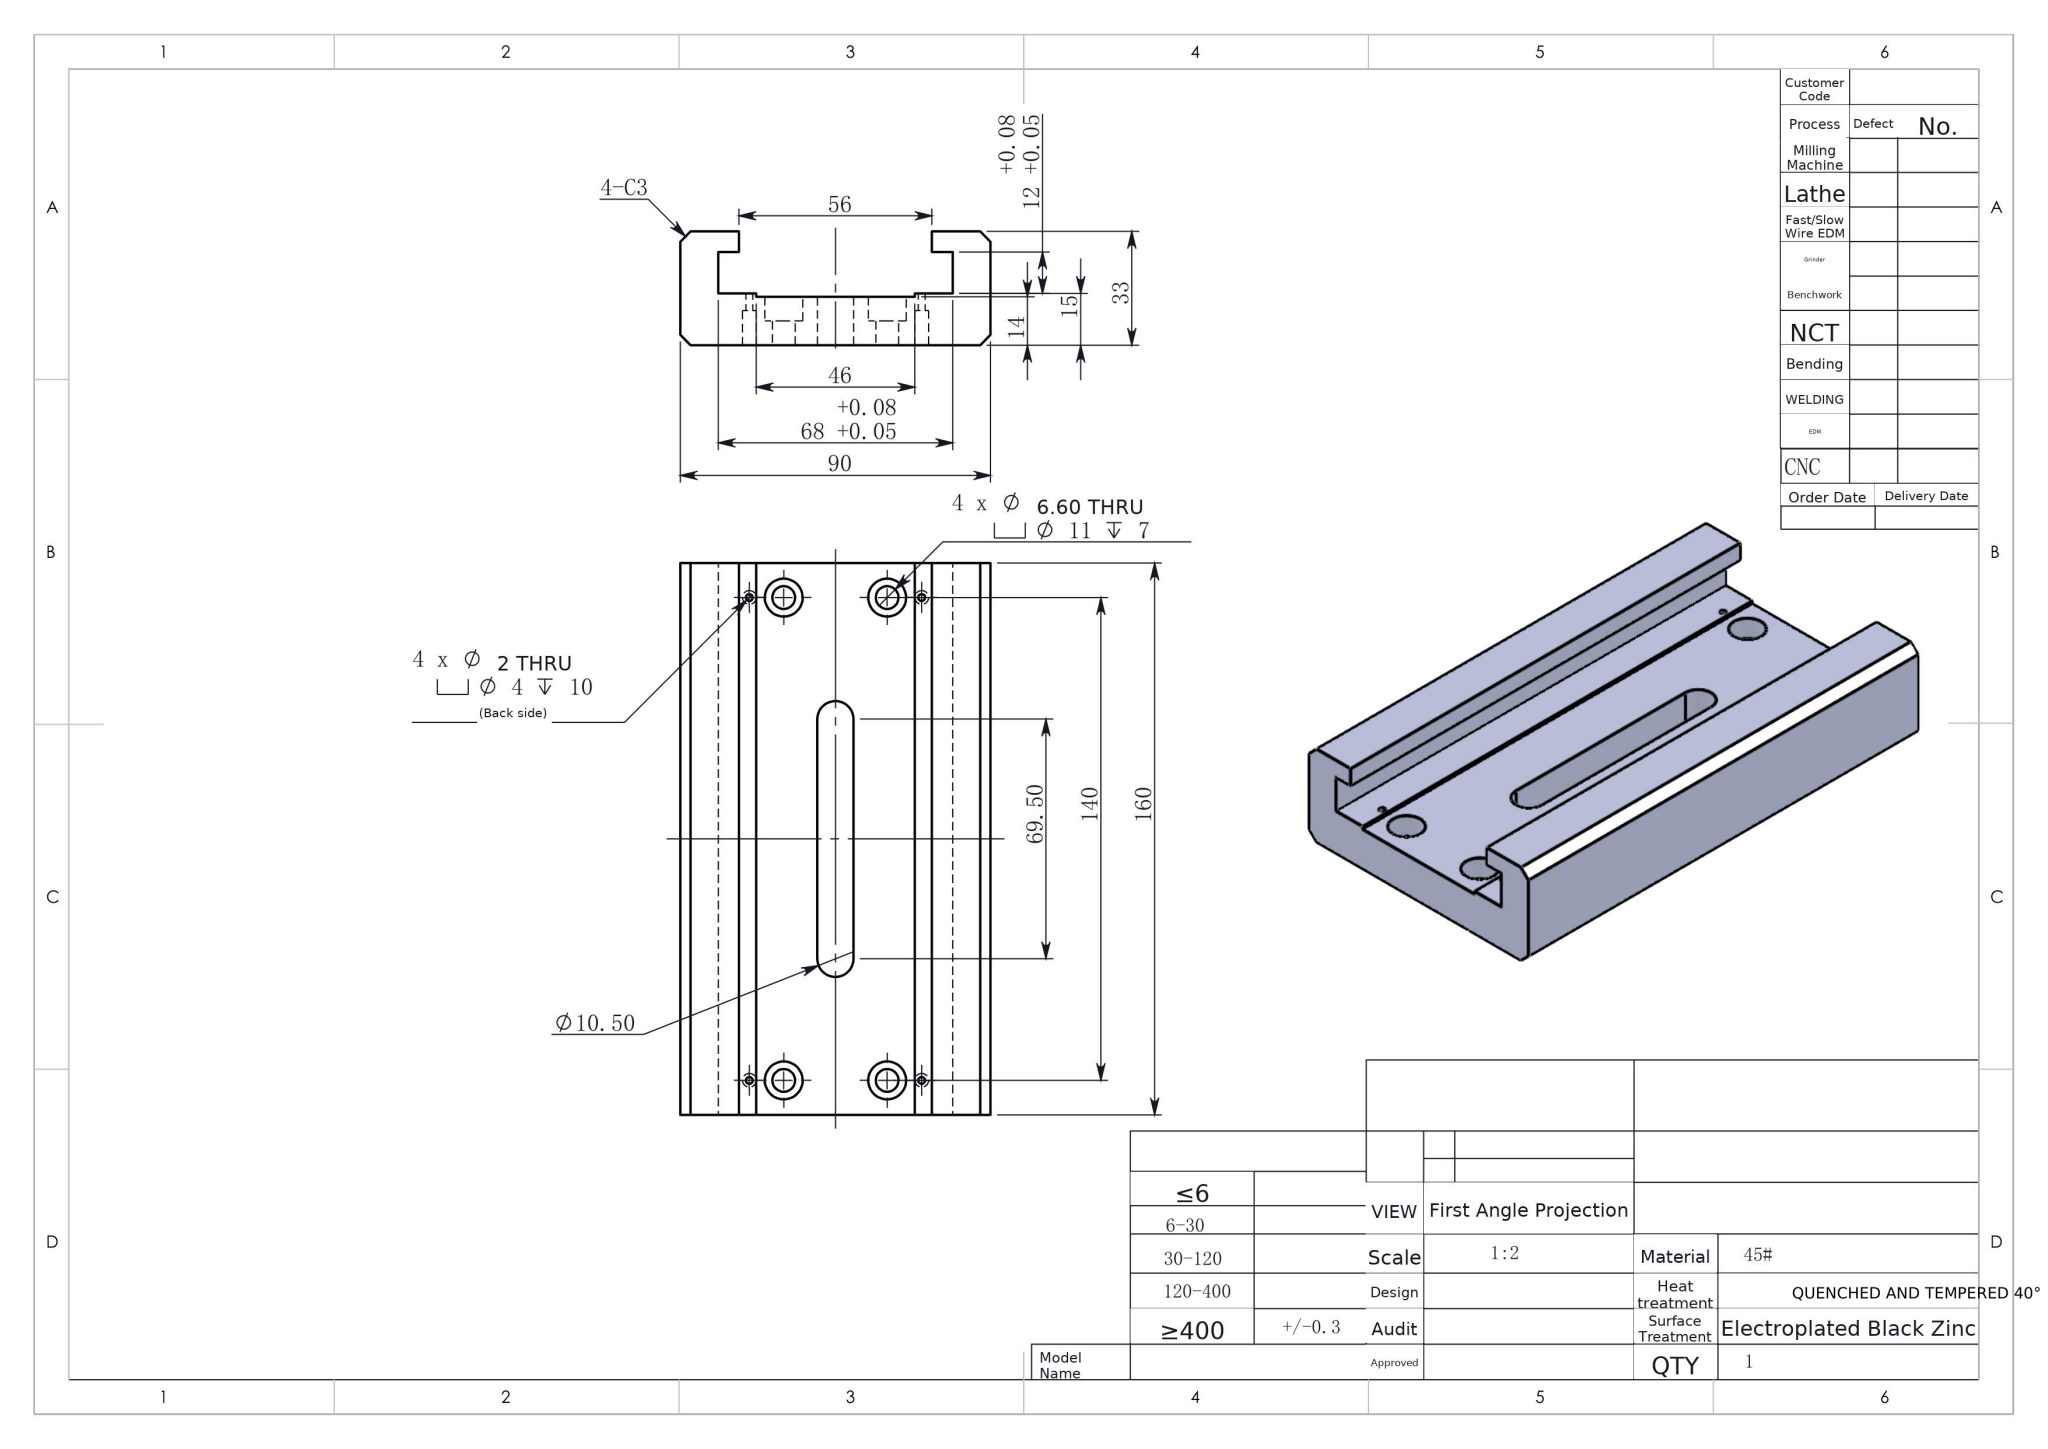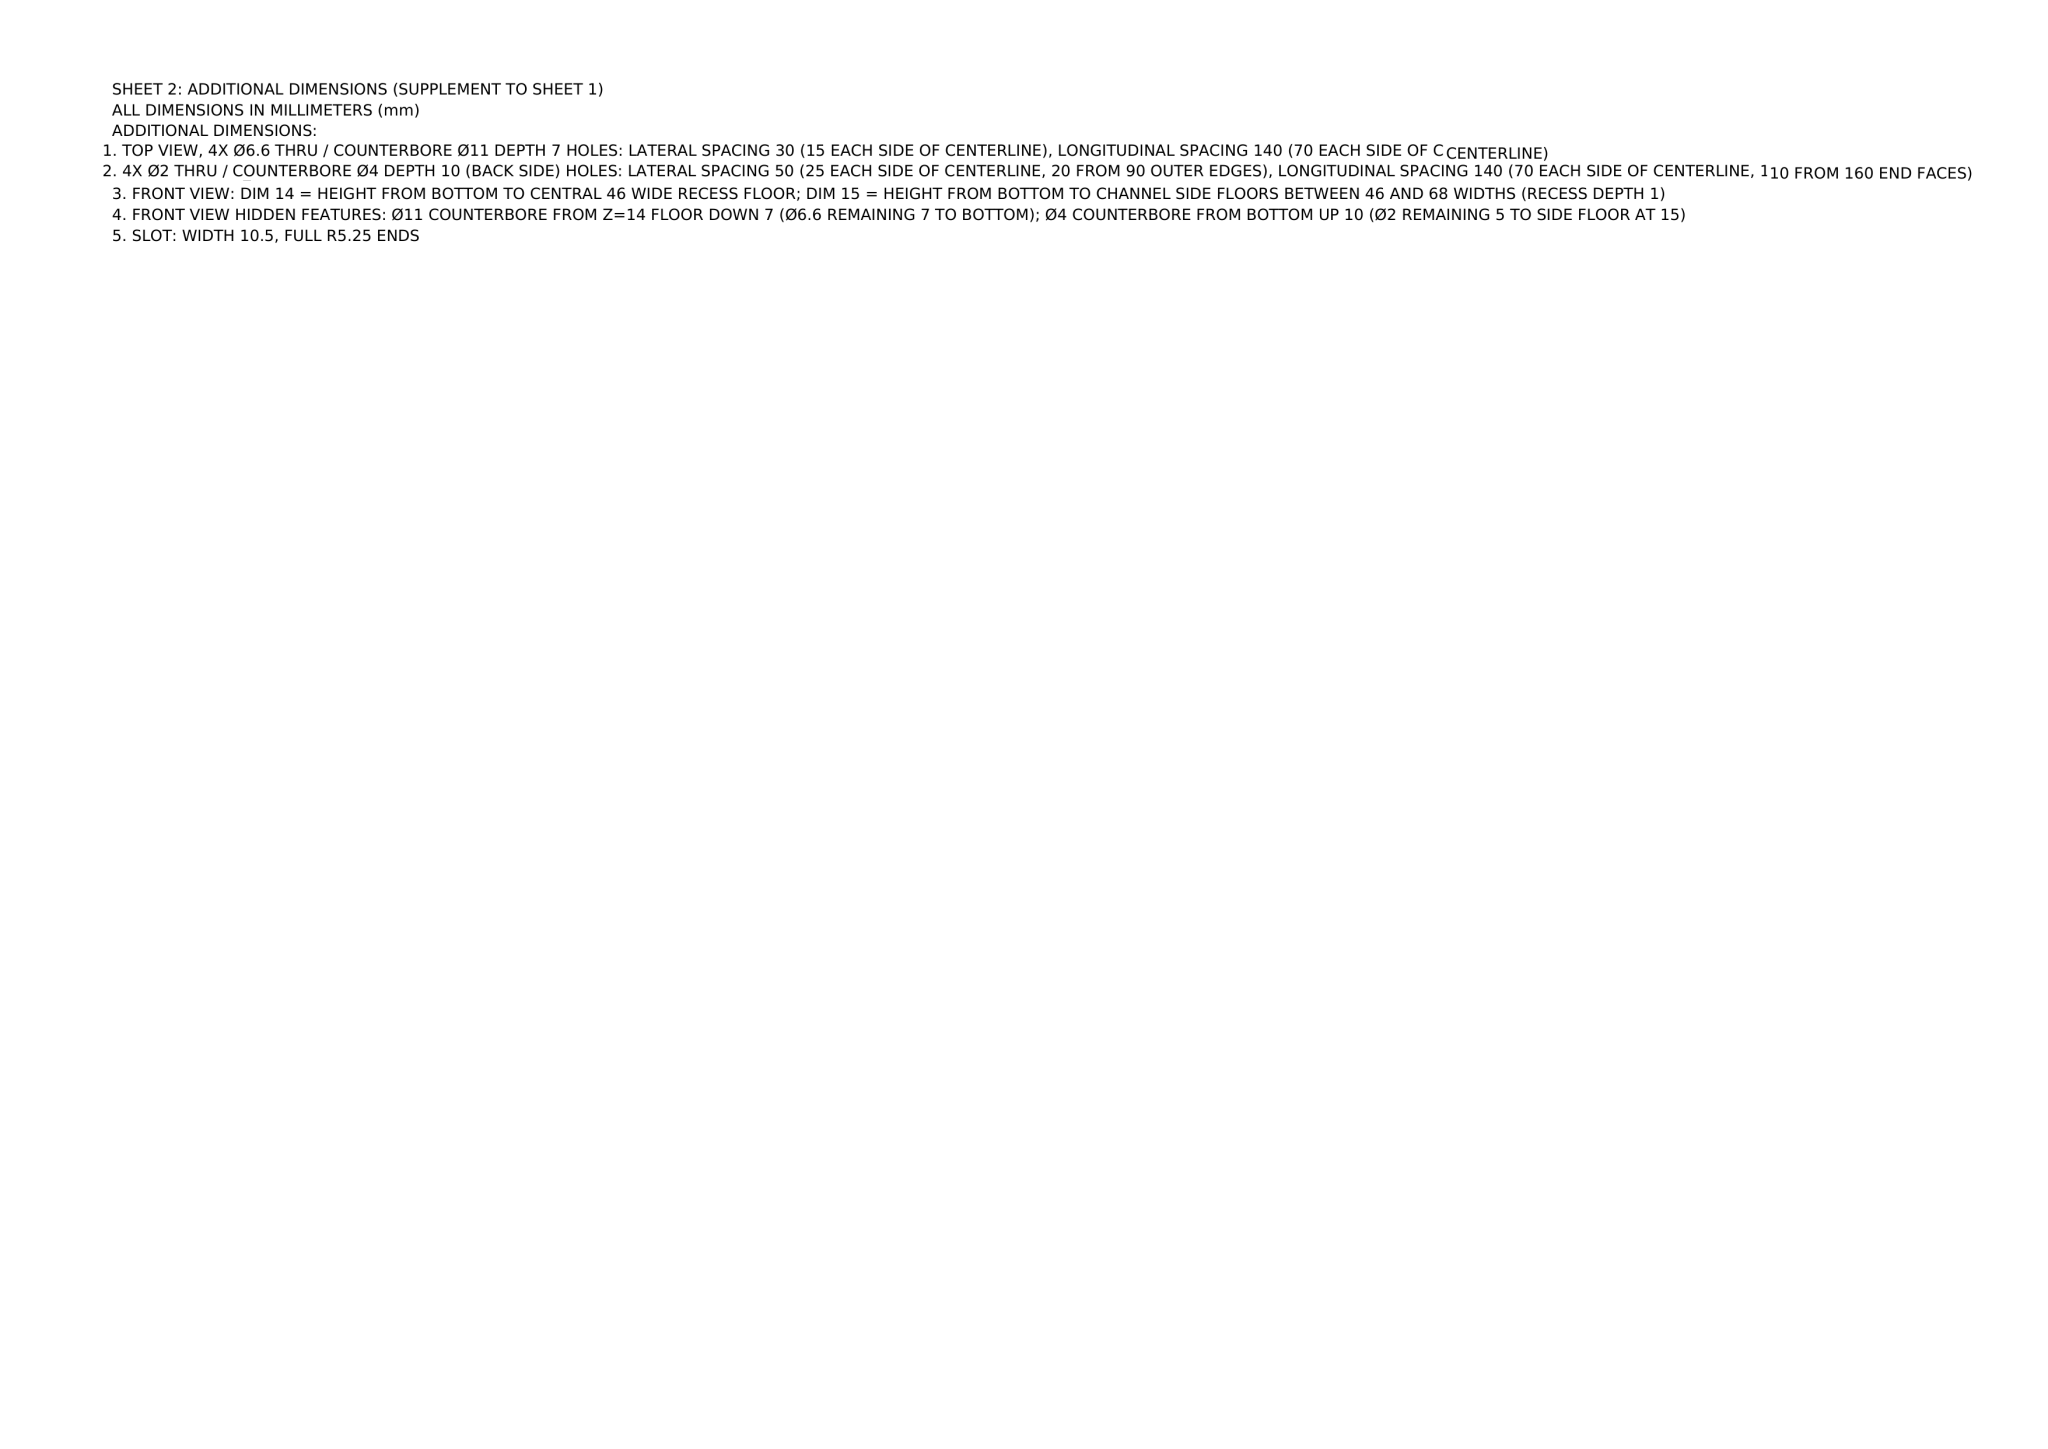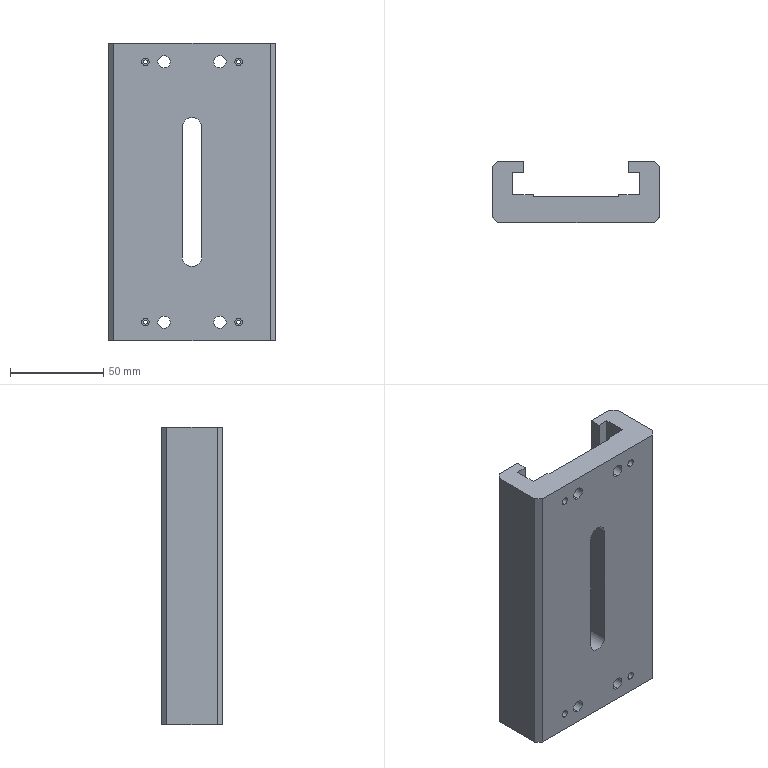Part | NX | mm | 1 solid | 67 faces | box 90 x 33 x 160 mm | volume 265027 mm3 | cylinder 35 | plane 32 | commonest cylinder face diameters 4 x8 2 x8 11 x8 6.6 x8 10.5 x3